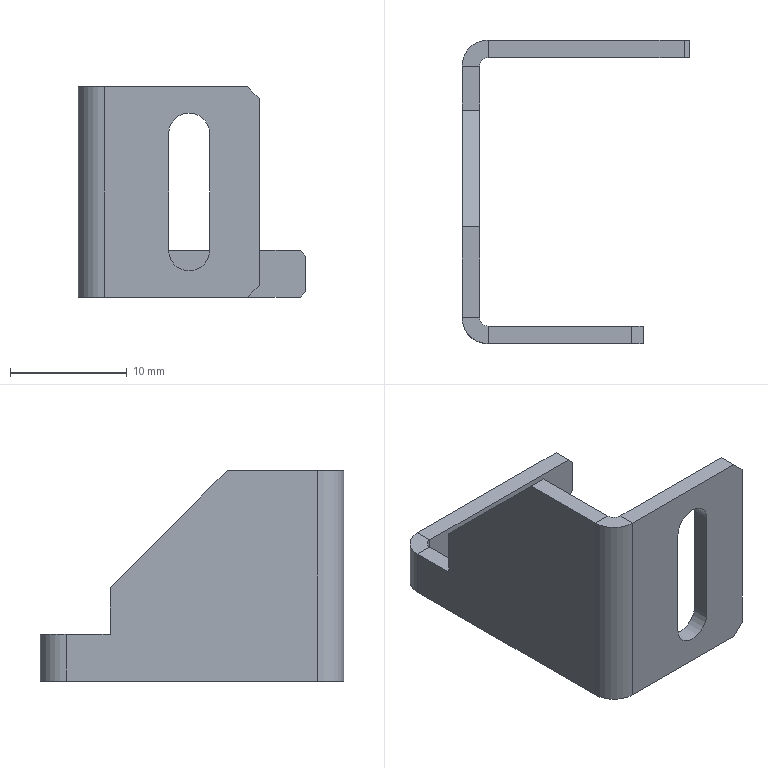Part | SolidWorks | mm | 1 solid | 34 faces | box 19.5 x 26 x 18 mm | volume 897 mm3 | plane 27 | cylinder 7 | commonest cylinder face diameters 3.5 x3 1.473 x2 4.473 x2
Drawing notes:
BOTH 90° BENDS: INSIDE R0.74, OUTSIDE R2.24 (1.5 THK) | from the solid: Z-axis cylinders dia 1.473 and 4.473 at (x2.24,y2.24) L18 and (x2.24,y23.76) L4; wall planes x0/x1.5 give 1.5 thk
2X C1 AT 15.50 FLANGE END, BOTH CORNERS (Z=0 & Z=18) | from the solid: Two inclined planes 45deg, size 1.0x1.5x1.0, at bbox_from [14.5,0,0] and [14.5,0,17] on the x=15.5 flange face (y 0-1.5, z 1-17)
STEP:
#1=CARTESIAN_POINT('',(8.,-1.5,15.75));
#2=VERTEX_POINT('',#1);
#3=CARTESIAN_POINT('',(9.75,-1.5,14.));
#4=VERTEX_POINT('',#3);
#5=CARTESIAN_POINT('',(8.,-1.5,14.));
#6=DIRECTION('',(0.,1.,0.));
#7=DIRECTION('',(0.,0.,1.));
#8=AXIS2_PLACEMENT_3D('',#5,#6,#7);
#9=CIRCLE('',#8,1.75);
#10=EDGE_CURVE('',#2,#4,#9,.T.);
#11=ORIENTED_EDGE('',*,*,#10,.F.);
#12=CARTESIAN_POINT('',(8.,0.,15.75));
#13=VERTEX_POINT('',#12);
#14=CARTESIAN_POINT('',(8.,-26.,15.75));
#15=DIRECTION('',(0.,1.,0.));
#16=VECTOR('',#15,1000.);
#17=LINE('',#14,#16);
#18=EDGE_CURVE('',#2,#13,#17,.T.);
#19=ORIENTED_EDGE('',*,*,#18,.T.);
#20=CARTESIAN_POINT('',(9.75,0.,14.));
#21=VERTEX_POINT('',#20);
#22=CARTESIAN_POINT('',(8.,0.,14.));
#23=DIRECTION('',(0.,1.,0.));
#24=DIRECTION('',(0.,0.,1.));
#25=AXIS2_PLACEMENT_3D('',#22,#23,#24);
#26=CIRCLE('',#25,1.75);
#27=EDGE_CURVE('',#13,#21,#26,.T.);
#28=ORIENTED_EDGE('',*,*,#27,.T.);
#29=CARTESIAN_POINT('',(9.75,-26.,14.));
#30=DIRECTION('',(0.,1.,0.));
#31=VECTOR('',#30,1000.);
#32=LINE('',#29,#31);
#33=EDGE_CURVE('',#4,#21,#32,.T.);
#34=ORIENTED_EDGE('',*,*,#33,.F.);
#35=EDGE_LOOP('',(#11,#19,#28,#34));
#36=FACE_OUTER_BOUND('',#35,.T.);
#37=CARTESIAN_POINT('',(8.,-26.,14.));
#38=DIRECTION('',(0.,1.,0.));
#39=DIRECTION('',(0.,0.,1.));
#40=AXIS2_PLACEMENT_3D('',#37,#38,#39);
#41=CYLINDRICAL_SURFACE('',#40,1.75);
#42=ADVANCED_FACE('',(#36),#41,.F.);
#43=CARTESIAN_POINT('',(0.7366,23.,4.));
#44=VERTEX_POINT('',#43);
#45=CARTESIAN_POINT('',(17.5,23.,4.));
#46=VERTEX_POINT('',#45);
#47=CARTESIAN_POINT('',(18.,23.,4.));
#48=DIRECTION('',(1.,0.,0.));
#49=VECTOR('',#48,1000.);
#50=LINE('',#47,#49);
#51=EDGE_CURVE('',#44,#46,#50,.T.);
#52=ORIENTED_EDGE('',*,*,#51,.T.);
#53=CARTESIAN_POINT('',(17.5,24.5,4.));
#54=VERTEX_POINT('',#53);
#55=CARTESIAN_POINT('',(17.5,24.5,4.));
#56=DIRECTION('',(0.,1.,0.));
#57=VECTOR('',#56,1000.);
#58=LINE('',#55,#57);
#59=EDGE_CURVE('',#46,#54,#58,.T.);
#60=ORIENTED_EDGE('',*,*,#59,.T.);
#61=CARTESIAN_POINT('',(0.7366,24.5,4.));
#62=VERTEX_POINT('',#61);
#63=CARTESIAN_POINT('',(18.,24.5,4.));
#64=DIRECTION('',(1.,0.,0.));
#65=VECTOR('',#64,1000.);
#66=LINE('',#63,#65);
#67=EDGE_CURVE('',#62,#54,#66,.T.);
#68=ORIENTED_EDGE('',*,*,#67,.F.);
#69=CARTESIAN_POINT('',(0.7366,24.5,4.));
#70=DIRECTION('',(-0.,-1.,0.));
#71=VECTOR('',#70,1000.);
#72=LINE('',#69,#71);
#73=EDGE_CURVE('',#62,#44,#72,.T.);
#74=ORIENTED_EDGE('',*,*,#73,.T.);
#75=EDGE_LOOP('',(#52,#60,#68,#74));
#76=FACE_OUTER_BOUND('',#75,.T.);
#77=CARTESIAN_POINT('',(24.5,30.5,4.));
#78=DIRECTION('',(0.,0.,-1.));
#79=DIRECTION('',(-1.,0.,0.));
#80=AXIS2_PLACEMENT_3D('',#77,#78,#79);
#81=PLANE('',#80);
#82=ADVANCED_FACE('',(#76),#81,.F.);
#83=CARTESIAN_POINT('',(0.,18.5,4.));
#84=VERTEX_POINT('',#83);
#85=CARTESIAN_POINT('',(0.,22.263,4.));
#86=VERTEX_POINT('',#85);
#87=CARTESIAN_POINT('',(0.,23.,4.));
#88=DIRECTION('',(0.,1.,0.));
#89=VECTOR('',#88,1000.);
#90=LINE('',#87,#89);
#91=EDGE_CURVE('',#84,#86,#90,.T.);
#92=ORIENTED_EDGE('',*,*,#91,.T.);
#93=CARTESIAN_POINT('',(-1.5,22.263,4.));
#94=VERTEX_POINT('',#93);
#95=CARTESIAN_POINT('',(0.,22.263,4.));
#96=DIRECTION('',(-1.,0.,0.));
#97=VECTOR('',#96,1000.);
#98=LINE('',#95,#97);
#99=EDGE_CURVE('',#86,#94,#98,.T.);
#100=ORIENTED_EDGE('',*,*,#99,.T.);
#101=CARTESIAN_POINT('',(-1.5,18.5,4.));
#102=VERTEX_POINT('',#101);
#103=CARTESIAN_POINT('',(-1.5,23.,4.));
#104=DIRECTION('',(0.,1.,0.));
#105=VECTOR('',#104,1000.);
#106=LINE('',#103,#105);
#107=EDGE_CURVE('',#102,#94,#106,.T.);
#108=ORIENTED_EDGE('',*,*,#107,.F.);
#109=CARTESIAN_POINT('',(24.5,18.5,4.));
#110=DIRECTION('',(-1.,0.,0.));
#111=VECTOR('',#110,1000.);
#112=LINE('',#109,#111);
#113=EDGE_CURVE('',#84,#102,#112,.T.);
#114=ORIENTED_EDGE('',*,*,#113,.F.);
#115=EDGE_LOOP('',(#92,#100,#108,#114));
#116=FACE_OUTER_BOUND('',#115,.T.);
#117=CARTESIAN_POINT('',(24.5,30.5,4.));
#118=DIRECTION('',(0.,0.,-1.));
#119=DIRECTION('',(-1.,0.,0.));
#120=AXIS2_PLACEMENT_3D('',#117,#118,#119);
#121=PLANE('',#120);
#122=ADVANCED_FACE('',(#116),#121,.F.);
#123=CARTESIAN_POINT('',(0.,8.5,18.));
#124=VERTEX_POINT('',#123);
#125=CARTESIAN_POINT('',(0.,0.7366,18.));
#126=VERTEX_POINT('',#125);
#127=CARTESIAN_POINT('',(0.,23.,18.));
#128=DIRECTION('',(-0.,-1.,0.));
#129=VECTOR('',#128,1000.);
#130=LINE('',#127,#129);
#131=EDGE_CURVE('',#124,#126,#130,.T.);
#132=ORIENTED_EDGE('',*,*,#131,.F.);
#133=CARTESIAN_POINT('',(-1.5,8.5,18.));
#134=VERTEX_POINT('',#133);
#135=CARTESIAN_POINT('',(-1.5,8.5,18.));
#136=DIRECTION('',(-1.,0.,0.));
#137=VECTOR('',#136,1000.);
#138=LINE('',#135,#137);
#139=EDGE_CURVE('',#124,#134,#138,.T.);
#140=ORIENTED_EDGE('',*,*,#139,.T.);
#141=CARTESIAN_POINT('',(-1.5,0.7366,18.));
#142=VERTEX_POINT('',#141);
#143=CARTESIAN_POINT('',(-1.5,23.,18.));
#144=DIRECTION('',(-0.,-1.,0.));
#145=VECTOR('',#144,1000.);
#146=LINE('',#143,#145);
#147=EDGE_CURVE('',#134,#142,#146,.T.);
#148=ORIENTED_EDGE('',*,*,#147,.T.);
#149=CARTESIAN_POINT('',(-1.5,0.7366,18.));
#150=DIRECTION('',(1.,-0.,0.));
#151=VECTOR('',#150,1000.);
#152=LINE('',#149,#151);
#153=EDGE_CURVE('',#142,#126,#152,.T.);
#154=ORIENTED_EDGE('',*,*,#153,.T.);
#155=EDGE_LOOP('',(#132,#140,#148,#154));
#156=FACE_OUTER_BOUND('',#155,.T.);
#157=CARTESIAN_POINT('',(0.7366,24.5,18.));
#158=DIRECTION('',(0.,0.,1.));
#159=DIRECTION('',(1.,0.,0.));
#160=AXIS2_PLACEMENT_3D('',#157,#158,#159);
#161=PLANE('',#160);
#162=ADVANCED_FACE('',(#156),#161,.T.);
#163=CARTESIAN_POINT('',(0.7366,23.,0.));
#164=VERTEX_POINT('',#163);
#165=CARTESIAN_POINT('',(0.7366,24.5,0.));
#166=VERTEX_POINT('',#165);
#167=CARTESIAN_POINT('',(0.7366,23.,0.));
#168=DIRECTION('',(0.,1.,0.));
#169=VECTOR('',#168,1000.);
#170=LINE('',#167,#169);
#171=EDGE_CURVE('',#164,#166,#170,.T.);
#172=ORIENTED_EDGE('',*,*,#171,.F.);
#173=CARTESIAN_POINT('',(0.,22.263,0.));
#174=VERTEX_POINT('',#173);
#175=CARTESIAN_POINT('',(0.7366,22.263,0.));
#176=DIRECTION('',(0.,0.,1.));
#177=DIRECTION('',(-1.,0.,0.));
#178=AXIS2_PLACEMENT_3D('',#175,#176,#177);
#179=CIRCLE('',#178,0.7366);
#180=EDGE_CURVE('',#164,#174,#179,.T.);
#181=ORIENTED_EDGE('',*,*,#180,.T.);
#182=CARTESIAN_POINT('',(-1.5,22.263,0.));
#183=VERTEX_POINT('',#182);
#184=CARTESIAN_POINT('',(-1.5,22.263,0.));
#185=DIRECTION('',(1.,0.,0.));
#186=VECTOR('',#185,1000.);
#187=LINE('',#184,#186);
#188=EDGE_CURVE('',#183,#174,#187,.T.);
#189=ORIENTED_EDGE('',*,*,#188,.F.);
#190=CARTESIAN_POINT('',(0.7366,22.263,0.));
#191=DIRECTION('',(0.,0.,1.));
#192=DIRECTION('',(1.,0.,0.));
#193=AXIS2_PLACEMENT_3D('',#190,#191,#192);
#194=CIRCLE('',#193,2.237);
#195=EDGE_CURVE('',#166,#183,#194,.T.);
#196=ORIENTED_EDGE('',*,*,#195,.F.);
#197=EDGE_LOOP('',(#172,#181,#189,#196));
#198=FACE_OUTER_BOUND('',#197,.T.);
#199=CARTESIAN_POINT('',(0.7366,23.,0.));
#200=DIRECTION('',(0.,0.,-1.));
#201=DIRECTION('',(-1.,0.,0.));
#202=AXIS2_PLACEMENT_3D('',#199,#200,#201);
#203=PLANE('',#202);
#204=ADVANCED_FACE('',(#198),#203,.T.);
#205=CARTESIAN_POINT('',(17.5,24.5,0.));
#206=VERTEX_POINT('',#205);
#207=CARTESIAN_POINT('',(18.,24.5,0.));
#208=DIRECTION('',(-1.,0.,0.));
#209=VECTOR('',#208,1000.);
#210=LINE('',#207,#209);
#211=EDGE_CURVE('',#206,#166,#210,.T.);
#212=ORIENTED_EDGE('',*,*,#211,.F.);
#213=CARTESIAN_POINT('',(17.5,23.,0.));
#214=VERTEX_POINT('',#213);
#215=CARTESIAN_POINT('',(17.5,22.263,0.));
#216=DIRECTION('',(0.,-1.,0.));
#217=VECTOR('',#216,1000.);
#218=LINE('',#215,#217);
#219=EDGE_CURVE('',#206,#214,#218,.T.);
#220=ORIENTED_EDGE('',*,*,#219,.T.);
#221=CARTESIAN_POINT('',(18.,23.,0.));
#222=DIRECTION('',(-1.,0.,0.));
#223=VECTOR('',#222,1000.);
#224=LINE('',#221,#223);
#225=EDGE_CURVE('',#214,#164,#224,.T.);
#226=ORIENTED_EDGE('',*,*,#225,.T.);
#227=ORIENTED_EDGE('',*,*,#171,.T.);
#228=EDGE_LOOP('',(#212,#220,#226,#227));
#229=FACE_OUTER_BOUND('',#228,.T.);
#230=CARTESIAN_POINT('',(-1.5,22.263,0.));
#231=DIRECTION('',(0.,0.,-1.));
#232=DIRECTION('',(-1.,0.,0.));
#233=AXIS2_PLACEMENT_3D('',#230,#231,#232);
#234=PLANE('',#233);
#235=ADVANCED_FACE('',(#229),#234,.T.);
#236=CARTESIAN_POINT('',(0.7366,0.,18.));
#237=VERTEX_POINT('',#236);
#238=CARTESIAN_POINT('',(0.7366,-1.5,18.));
#239=VERTEX_POINT('',#238);
#240=CARTESIAN_POINT('',(0.7366,0.,18.));
#241=DIRECTION('',(0.,-1.,0.));
#242=VECTOR('',#241,1000.);
#243=LINE('',#240,#242);
#244=EDGE_CURVE('',#237,#239,#243,.T.);
#245=ORIENTED_EDGE('',*,*,#244,.F.);
#246=CARTESIAN_POINT('',(0.7366,0.7366,18.));
#247=DIRECTION('',(0.,0.,1.));
#248=DIRECTION('',(-1.,0.,0.));
#249=AXIS2_PLACEMENT_3D('',#246,#247,#248);
#250=CIRCLE('',#249,0.7366);
#251=EDGE_CURVE('',#126,#237,#250,.T.);
#252=ORIENTED_EDGE('',*,*,#251,.F.);
#253=ORIENTED_EDGE('',*,*,#153,.F.);
#254=CARTESIAN_POINT('',(0.7366,0.7366,18.));
#255=DIRECTION('',(0.,0.,1.));
#256=DIRECTION('',(1.,0.,0.));
#257=AXIS2_PLACEMENT_3D('',#254,#255,#256);
#258=CIRCLE('',#257,2.237);
#259=EDGE_CURVE('',#142,#239,#258,.T.);
#260=ORIENTED_EDGE('',*,*,#259,.T.);
#261=EDGE_LOOP('',(#245,#252,#253,#260));
#262=FACE_OUTER_BOUND('',#261,.T.);
#263=CARTESIAN_POINT('',(0.7366,0.,18.));
#264=DIRECTION('',(0.,0.,1.));
#265=DIRECTION('',(1.,0.,0.));
#266=AXIS2_PLACEMENT_3D('',#263,#264,#265);
#267=PLANE('',#266);
#268=ADVANCED_FACE('',(#262),#267,.T.);
#269=CARTESIAN_POINT('',(13.,-1.5,18.));
#270=VERTEX_POINT('',#269);
#271=CARTESIAN_POINT('',(0.,-1.5,18.));
#272=DIRECTION('',(1.,0.,0.));
#273=VECTOR('',#272,1000.);
#274=LINE('',#271,#273);
#275=EDGE_CURVE('',#239,#270,#274,.T.);
#276=ORIENTED_EDGE('',*,*,#275,.T.);
#277=CARTESIAN_POINT('',(13.,0.,18.));
#278=VERTEX_POINT('',#277);
#279=CARTESIAN_POINT('',(13.,0.7366,18.));
#280=DIRECTION('',(0.,1.,0.));
#281=VECTOR('',#280,1000.);
#282=LINE('',#279,#281);
#283=EDGE_CURVE('',#270,#278,#282,.T.);
#284=ORIENTED_EDGE('',*,*,#283,.T.);
#285=CARTESIAN_POINT('',(0.,0.,18.));
#286=DIRECTION('',(1.,0.,0.));
#287=VECTOR('',#286,1000.);
#288=LINE('',#285,#287);
#289=EDGE_CURVE('',#237,#278,#288,.T.);
#290=ORIENTED_EDGE('',*,*,#289,.F.);
#291=ORIENTED_EDGE('',*,*,#244,.T.);
#292=EDGE_LOOP('',(#276,#284,#290,#291));
#293=FACE_OUTER_BOUND('',#292,.T.);
#294=CARTESIAN_POINT('',(-1.5,0.7366,18.));
#295=DIRECTION('',(0.,0.,1.));
#296=DIRECTION('',(1.,0.,0.));
#297=AXIS2_PLACEMENT_3D('',#294,#295,#296);
#298=PLANE('',#297);
#299=ADVANCED_FACE('',(#293),#298,.T.);
#300=CARTESIAN_POINT('',(0.,0.7366,0.));
#301=VERTEX_POINT('',#300);
#302=CARTESIAN_POINT('',(-1.5,0.7366,0.));
#303=VERTEX_POINT('',#302);
#304=CARTESIAN_POINT('',(0.,0.7366,0.));
#305=DIRECTION('',(-1.,0.,0.));
#306=VECTOR('',#305,1000.);
#307=LINE('',#304,#306);
#308=EDGE_CURVE('',#301,#303,#307,.T.);
#309=ORIENTED_EDGE('',*,*,#308,.F.);
#310=CARTESIAN_POINT('',(0.7366,0.,0.));
#311=VERTEX_POINT('',#310);
#312=CARTESIAN_POINT('',(0.7366,0.7366,0.));
#313=DIRECTION('',(0.,0.,1.));
#314=DIRECTION('',(-1.,0.,0.));
#315=AXIS2_PLACEMENT_3D('',#312,#313,#314);
#316=CIRCLE('',#315,0.7366);
#317=EDGE_CURVE('',#301,#311,#316,.T.);
#318=ORIENTED_EDGE('',*,*,#317,.T.);
#319=CARTESIAN_POINT('',(0.7366,-1.5,0.));
#320=VERTEX_POINT('',#319);
#321=CARTESIAN_POINT('',(0.7366,-1.5,0.));
#322=DIRECTION('',(0.,1.,0.));
#323=VECTOR('',#322,1000.);
#324=LINE('',#321,#323);
#325=EDGE_CURVE('',#320,#311,#324,.T.);
#326=ORIENTED_EDGE('',*,*,#325,.F.);
#327=CARTESIAN_POINT('',(0.7366,0.7366,0.));
#328=DIRECTION('',(0.,0.,1.));
#329=DIRECTION('',(1.,0.,0.));
#330=AXIS2_PLACEMENT_3D('',#327,#328,#329);
#331=CIRCLE('',#330,2.237);
#332=EDGE_CURVE('',#303,#320,#331,.T.);
#333=ORIENTED_EDGE('',*,*,#332,.F.);
#334=EDGE_LOOP('',(#309,#318,#326,#333));
#335=FACE_OUTER_BOUND('',#334,.T.);
#336=CARTESIAN_POINT('',(0.,0.7366,0.));
#337=DIRECTION('',(0.,0.,-1.));
#338=DIRECTION('',(-1.,0.,0.));
#339=AXIS2_PLACEMENT_3D('',#336,#337,#338);
#340=PLANE('',#339);
#341=ADVANCED_FACE('',(#335),#340,.T.);
#342=CARTESIAN_POINT('',(0.,23.,0.));
#343=DIRECTION('',(-0.,-1.,0.));
#344=VECTOR('',#343,1000.);
#345=LINE('',#342,#344);
#346=EDGE_CURVE('',#174,#301,#345,.T.);
#347=ORIENTED_EDGE('',*,*,#346,.T.);
#348=ORIENTED_EDGE('',*,*,#308,.T.);
#349=CARTESIAN_POINT('',(-1.5,23.,0.));
#350=DIRECTION('',(-0.,-1.,0.));
#351=VECTOR('',#350,1000.);
#352=LINE('',#349,#351);
#353=EDGE_CURVE('',#183,#303,#352,.T.);
#354=ORIENTED_EDGE('',*,*,#353,.F.);
#355=ORIENTED_EDGE('',*,*,#188,.T.);
#356=EDGE_LOOP('',(#347,#348,#354,#355));
#357=FACE_OUTER_BOUND('',#356,.T.);
#358=CARTESIAN_POINT('',(0.7366,-1.5,0.));
#359=DIRECTION('',(0.,0.,-1.));
#360=DIRECTION('',(-1.,0.,0.));
#361=AXIS2_PLACEMENT_3D('',#358,#359,#360);
#362=PLANE('',#361);
#363=ADVANCED_FACE('',(#357),#362,.T.);
#364=CARTESIAN_POINT('',(6.25,-1.5,4.));
#365=VERTEX_POINT('',#364);
#366=CARTESIAN_POINT('',(6.25,-1.5,14.));
#367=VERTEX_POINT('',#366);
#368=CARTESIAN_POINT('',(6.25,-1.5,18.));
#369=DIRECTION('',(0.,0.,1.));
#370=VECTOR('',#369,1000.);
#371=LINE('',#368,#370);
#372=EDGE_CURVE('',#365,#367,#371,.T.);
#373=ORIENTED_EDGE('',*,*,#372,.T.);
#374=CARTESIAN_POINT('',(8.,-1.5,14.));
#375=DIRECTION('',(0.,1.,0.));
#376=DIRECTION('',(0.,0.,1.));
#377=AXIS2_PLACEMENT_3D('',#374,#375,#376);
#378=CIRCLE('',#377,1.75);
#379=EDGE_CURVE('',#367,#2,#378,.T.);
#380=ORIENTED_EDGE('',*,*,#379,.T.);
#381=ORIENTED_EDGE('',*,*,#10,.T.);
#382=CARTESIAN_POINT('',(9.75,-1.5,4.));
#383=VERTEX_POINT('',#382);
#384=CARTESIAN_POINT('',(9.75,-1.5,18.));
#385=DIRECTION('',(0.,0.,-1.));
#386=VECTOR('',#385,1000.);
#387=LINE('',#384,#386);
#388=EDGE_CURVE('',#4,#383,#387,.T.);
#389=ORIENTED_EDGE('',*,*,#388,.T.);
#390=CARTESIAN_POINT('',(8.,-1.5,4.));
#391=DIRECTION('',(0.,1.,0.));
#392=DIRECTION('',(0.,0.,1.));
#393=AXIS2_PLACEMENT_3D('',#390,#391,#392);
#394=CIRCLE('',#393,1.75);
#395=EDGE_CURVE('',#383,#365,#394,.T.);
#396=ORIENTED_EDGE('',*,*,#395,.T.);
#397=EDGE_LOOP('',(#373,#380,#381,#389,#396));
#398=FACE_BOUND('',#397,.T.);
#399=CARTESIAN_POINT('',(13.,-1.5,0.));
#400=VERTEX_POINT('',#399);
#401=CARTESIAN_POINT('',(0.,-1.5,0.));
#402=DIRECTION('',(1.,0.,0.));
#403=VECTOR('',#402,1000.);
#404=LINE('',#401,#403);
#405=EDGE_CURVE('',#320,#400,#404,.T.);
#406=ORIENTED_EDGE('',*,*,#405,.T.);
#407=CARTESIAN_POINT('',(14.,-1.5,1.));
#408=VERTEX_POINT('',#407);
#409=CARTESIAN_POINT('',(13.,-1.5,0.));
#410=DIRECTION('',(0.7071,0.,0.7071));
#411=VECTOR('',#410,1000.);
#412=LINE('',#409,#411);
#413=EDGE_CURVE('',#400,#408,#412,.T.);
#414=ORIENTED_EDGE('',*,*,#413,.T.);
#415=CARTESIAN_POINT('',(14.,-1.5,17.));
#416=VERTEX_POINT('',#415);
#417=CARTESIAN_POINT('',(14.,-1.5,18.));
#418=DIRECTION('',(0.,0.,-1.));
#419=VECTOR('',#418,1000.);
#420=LINE('',#417,#419);
#421=EDGE_CURVE('',#416,#408,#420,.T.);
#422=ORIENTED_EDGE('',*,*,#421,.F.);
#423=CARTESIAN_POINT('',(14.,-1.5,17.));
#424=DIRECTION('',(-0.7071,0.,0.7071));
#425=VECTOR('',#424,1000.);
#426=LINE('',#423,#425);
#427=EDGE_CURVE('',#416,#270,#426,.T.);
#428=ORIENTED_EDGE('',*,*,#427,.T.);
#429=ORIENTED_EDGE('',*,*,#275,.F.);
#430=CARTESIAN_POINT('',(0.7366,-1.5,18.));
#431=DIRECTION('',(0.,0.,-1.));
#432=VECTOR('',#431,1000.);
#433=LINE('',#430,#432);
#434=EDGE_CURVE('',#239,#320,#433,.T.);
#435=ORIENTED_EDGE('',*,*,#434,.T.);
#436=EDGE_LOOP('',(#406,#414,#422,#428,#429,#435));
#437=FACE_OUTER_BOUND('',#436,.T.);
#438=CARTESIAN_POINT('',(0.,-1.5,18.));
#439=DIRECTION('',(0.,1.,0.));
#440=DIRECTION('',(0.,0.,1.));
#441=AXIS2_PLACEMENT_3D('',#438,#439,#440);
#442=PLANE('',#441);
#443=ADVANCED_FACE('',(#398,#437),#442,.F.);
#444=ORIENTED_EDGE('',*,*,#421,.T.);
#445=CARTESIAN_POINT('',(14.,0.,1.));
#446=VERTEX_POINT('',#445);
#447=CARTESIAN_POINT('',(14.,0.,1.));
#448=DIRECTION('',(0.,1.,0.));
#449=VECTOR('',#448,1000.);
#450=LINE('',#447,#449);
#451=EDGE_CURVE('',#408,#446,#450,.T.);
#452=ORIENTED_EDGE('',*,*,#451,.T.);
#453=CARTESIAN_POINT('',(14.,0.,17.));
#454=VERTEX_POINT('',#453);
#455=CARTESIAN_POINT('',(14.,0.,18.));
#456=DIRECTION('',(0.,0.,-1.));
#457=VECTOR('',#456,1000.);
#458=LINE('',#455,#457);
#459=EDGE_CURVE('',#454,#446,#458,.T.);
#460=ORIENTED_EDGE('',*,*,#459,.F.);
#461=CARTESIAN_POINT('',(14.,0.,17.));
#462=DIRECTION('',(0.,-1.,0.));
#463=VECTOR('',#462,1000.);
#464=LINE('',#461,#463);
#465=EDGE_CURVE('',#454,#416,#464,.T.);
#466=ORIENTED_EDGE('',*,*,#465,.T.);
#467=EDGE_LOOP('',(#444,#452,#460,#466));
#468=FACE_OUTER_BOUND('',#467,.T.);
#469=CARTESIAN_POINT('',(14.,0.,18.));
#470=DIRECTION('',(1.,0.,0.));
#471=DIRECTION('',(0.,0.,-1.));
#472=AXIS2_PLACEMENT_3D('',#469,#470,#471);
#473=PLANE('',#472);
#474=ADVANCED_FACE('',(#468),#473,.T.);
#475=CARTESIAN_POINT('',(6.25,0.,14.));
#476=VERTEX_POINT('',#475);
#477=CARTESIAN_POINT('',(8.,0.,14.));
#478=DIRECTION('',(0.,1.,0.));
#479=DIRECTION('',(0.,0.,1.));
#480=AXIS2_PLACEMENT_3D('',#477,#478,#479);
#481=CIRCLE('',#480,1.75);
#482=EDGE_CURVE('',#476,#13,#481,.T.);
#483=ORIENTED_EDGE('',*,*,#482,.F.);
#484=CARTESIAN_POINT('',(6.25,0.,4.));
#485=VERTEX_POINT('',#484);
#486=CARTESIAN_POINT('',(6.25,0.,14.));
#487=DIRECTION('',(0.,0.,1.));
#488=VECTOR('',#487,1000.);
#489=LINE('',#486,#488);
#490=EDGE_CURVE('',#485,#476,#489,.T.);
#491=ORIENTED_EDGE('',*,*,#490,.F.);
#492=CARTESIAN_POINT('',(9.75,0.,4.));
#493=VERTEX_POINT('',#492);
#494=CARTESIAN_POINT('',(8.,0.,4.));
#495=DIRECTION('',(0.,1.,0.));
#496=DIRECTION('',(0.,0.,1.));
#497=AXIS2_PLACEMENT_3D('',#494,#495,#496);
#498=CIRCLE('',#497,1.75);
#499=EDGE_CURVE('',#493,#485,#498,.T.);
#500=ORIENTED_EDGE('',*,*,#499,.F.);
#501=CARTESIAN_POINT('',(9.75,0.,14.));
#502=DIRECTION('',(0.,0.,-1.));
#503=VECTOR('',#502,1000.);
#504=LINE('',#501,#503);
#505=EDGE_CURVE('',#21,#493,#504,.T.);
#506=ORIENTED_EDGE('',*,*,#505,.F.);
#507=ORIENTED_EDGE('',*,*,#27,.F.);
#508=EDGE_LOOP('',(#483,#491,#500,#506,#507));
#509=FACE_BOUND('',#508,.T.);
#510=ORIENTED_EDGE('',*,*,#459,.T.);
#511=CARTESIAN_POINT('',(13.,0.,0.));
#512=VERTEX_POINT('',#511);
#513=CARTESIAN_POINT('',(15.5,0.,2.5));
#514=DIRECTION('',(-0.7071,0.,-0.7071));
#515=VECTOR('',#514,1000.);
#516=LINE('',#513,#515);
#517=EDGE_CURVE('',#446,#512,#516,.T.);
#518=ORIENTED_EDGE('',*,*,#517,.T.);
#519=CARTESIAN_POINT('',(0.,0.,0.));
#520=DIRECTION('',(1.,0.,0.));
#521=VECTOR('',#520,1000.);
#522=LINE('',#519,#521);
#523=EDGE_CURVE('',#311,#512,#522,.T.);
#524=ORIENTED_EDGE('',*,*,#523,.F.);
#525=CARTESIAN_POINT('',(0.7366,0.,18.));
#526=DIRECTION('',(0.,0.,-1.));
#527=VECTOR('',#526,1000.);
#528=LINE('',#525,#527);
#529=EDGE_CURVE('',#237,#311,#528,.T.);
#530=ORIENTED_EDGE('',*,*,#529,.F.);
#531=ORIENTED_EDGE('',*,*,#289,.T.);
#532=CARTESIAN_POINT('',(6.5,0.,24.5));
#533=DIRECTION('',(0.7071,0.,-0.7071));
#534=VECTOR('',#533,1000.);
#535=LINE('',#532,#534);
#536=EDGE_CURVE('',#278,#454,#535,.T.);
#537=ORIENTED_EDGE('',*,*,#536,.T.);
#538=EDGE_LOOP('',(#510,#518,#524,#530,#531,#537));
#539=FACE_OUTER_BOUND('',#538,.T.);
#540=CARTESIAN_POINT('',(0.,0.,18.));
#541=DIRECTION('',(0.,1.,0.));
#542=DIRECTION('',(0.,0.,1.));
#543=AXIS2_PLACEMENT_3D('',#540,#541,#542);
#544=PLANE('',#543);
#545=ADVANCED_FACE('',(#509,#539),#544,.T.);
#546=ORIENTED_EDGE('',*,*,#317,.F.);
#547=CARTESIAN_POINT('',(0.,0.7366,18.));
#548=DIRECTION('',(0.,0.,-1.));
#549=VECTOR('',#548,1000.);
#550=LINE('',#547,#549);
#551=EDGE_CURVE('',#126,#301,#550,.T.);
#552=ORIENTED_EDGE('',*,*,#551,.F.);
#553=ORIENTED_EDGE('',*,*,#251,.T.);
#554=ORIENTED_EDGE('',*,*,#529,.T.);
#555=EDGE_LOOP('',(#546,#552,#553,#554));
#556=FACE_OUTER_BOUND('',#555,.T.);
#557=CARTESIAN_POINT('',(0.7366,0.7366,18.));
#558=DIRECTION('',(0.,0.,-1.));
#559=DIRECTION('',(-1.,0.,0.));
#560=AXIS2_PLACEMENT_3D('',#557,#558,#559);
#561=CYLINDRICAL_SURFACE('',#560,0.7366);
#562=ADVANCED_FACE('',(#556),#561,.F.);
#563=CARTESIAN_POINT('',(0.,18.5,8.));
#564=VERTEX_POINT('',#563);
#565=CARTESIAN_POINT('',(0.,18.5,18.));
#566=DIRECTION('',(0.,0.,-1.));
#567=VECTOR('',#566,1000.);
#568=LINE('',#565,#567);
#569=EDGE_CURVE('',#564,#84,#568,.T.);
#570=ORIENTED_EDGE('',*,*,#569,.F.);
#571=CARTESIAN_POINT('',(0.,15.75,10.75));
#572=DIRECTION('',(-0.,-0.7071,0.7071));
#573=VECTOR('',#572,1000.);
#574=LINE('',#571,#573);
#575=EDGE_CURVE('',#564,#124,#574,.T.);
#576=ORIENTED_EDGE('',*,*,#575,.T.);
#577=ORIENTED_EDGE('',*,*,#131,.T.);
#578=ORIENTED_EDGE('',*,*,#551,.T.);
#579=ORIENTED_EDGE('',*,*,#346,.F.);
#580=CARTESIAN_POINT('',(0.,22.263,18.));
#581=DIRECTION('',(0.,0.,-1.));
#582=VECTOR('',#581,1000.);
#583=LINE('',#580,#582);
#584=EDGE_CURVE('',#86,#174,#583,.T.);
#585=ORIENTED_EDGE('',*,*,#584,.F.);
#586=ORIENTED_EDGE('',*,*,#91,.F.);
#587=EDGE_LOOP('',(#570,#576,#577,#578,#579,#585,#586));
#588=FACE_OUTER_BOUND('',#587,.T.);
#589=CARTESIAN_POINT('',(0.,23.,18.));
#590=DIRECTION('',(1.,-0.,0.));
#591=DIRECTION('',(0.,1.,0.));
#592=AXIS2_PLACEMENT_3D('',#589,#590,#591);
#593=PLANE('',#592);
#594=ADVANCED_FACE('',(#588),#593,.T.);
#595=CARTESIAN_POINT('',(0.7366,22.263,4.));
#596=DIRECTION('',(0.,0.,-1.));
#597=DIRECTION('',(-1.,0.,0.));
#598=AXIS2_PLACEMENT_3D('',#595,#596,#597);
#599=CIRCLE('',#598,0.7366);
#600=EDGE_CURVE('',#86,#44,#599,.T.);
#601=ORIENTED_EDGE('',*,*,#600,.F.);
#602=ORIENTED_EDGE('',*,*,#584,.T.);
#603=ORIENTED_EDGE('',*,*,#180,.F.);
#604=CARTESIAN_POINT('',(0.7366,23.,18.));
#605=DIRECTION('',(0.,0.,-1.));
#606=VECTOR('',#605,1000.);
#607=LINE('',#604,#606);
#608=EDGE_CURVE('',#44,#164,#607,.T.);
#609=ORIENTED_EDGE('',*,*,#608,.F.);
#610=EDGE_LOOP('',(#601,#602,#603,#609));
#611=FACE_OUTER_BOUND('',#610,.T.);
#612=CARTESIAN_POINT('',(0.7366,22.263,18.));
#613=DIRECTION('',(0.,0.,-1.));
#614=DIRECTION('',(-1.,0.,0.));
#615=AXIS2_PLACEMENT_3D('',#612,#613,#614);
#616=CYLINDRICAL_SURFACE('',#615,0.7366);
#617=ADVANCED_FACE('',(#611),#616,.F.);
#618=CARTESIAN_POINT('',(18.,23.,3.5));
#619=VERTEX_POINT('',#618);
#620=CARTESIAN_POINT('',(18.,23.,0.5));
#621=VERTEX_POINT('',#620);
#622=CARTESIAN_POINT('',(18.,23.,18.));
#623=DIRECTION('',(0.,0.,-1.));
#624=VECTOR('',#623,1000.);
#625=LINE('',#622,#624);
#626=EDGE_CURVE('',#619,#621,#625,.T.);
#627=ORIENTED_EDGE('',*,*,#626,.F.);
#628=CARTESIAN_POINT('',(10.75,23.,10.75));
#629=DIRECTION('',(-0.7071,0.,0.7071));
#630=VECTOR('',#629,1000.);
#631=LINE('',#628,#630);
#632=EDGE_CURVE('',#619,#46,#631,.T.);
#633=ORIENTED_EDGE('',*,*,#632,.T.);
#634=ORIENTED_EDGE('',*,*,#51,.F.);
#635=ORIENTED_EDGE('',*,*,#608,.T.);
#636=ORIENTED_EDGE('',*,*,#225,.F.);
#637=CARTESIAN_POINT('',(26.75,23.,9.25));
#638=DIRECTION('',(0.7071,0.,0.7071));
#639=VECTOR('',#638,1000.);
#640=LINE('',#637,#639);
#641=EDGE_CURVE('',#214,#621,#640,.T.);
#642=ORIENTED_EDGE('',*,*,#641,.T.);
#643=EDGE_LOOP('',(#627,#633,#634,#635,#636,#642));
#644=FACE_OUTER_BOUND('',#643,.T.);
#645=CARTESIAN_POINT('',(18.,23.,18.));
#646=DIRECTION('',(0.,-1.,0.));
#647=DIRECTION('',(0.,0.,-1.));
#648=AXIS2_PLACEMENT_3D('',#645,#646,#647);
#649=PLANE('',#648);
#650=ADVANCED_FACE('',(#644),#649,.T.);
#651=CARTESIAN_POINT('',(18.,24.5,3.5));
#652=VERTEX_POINT('',#651);
#653=CARTESIAN_POINT('',(18.,24.5,0.5));
#654=VERTEX_POINT('',#653);
#655=CARTESIAN_POINT('',(18.,24.5,18.));
#656=DIRECTION('',(0.,0.,-1.));
#657=VECTOR('',#656,1000.);
#658=LINE('',#655,#657);
#659=EDGE_CURVE('',#652,#654,#658,.T.);
#660=ORIENTED_EDGE('',*,*,#659,.F.);
#661=CARTESIAN_POINT('',(18.,23.,3.5));
#662=DIRECTION('',(0.,-1.,0.));
#663=VECTOR('',#662,1000.);
#664=LINE('',#661,#663);
#665=EDGE_CURVE('',#652,#619,#664,.T.);
#666=ORIENTED_EDGE('',*,*,#665,.T.);
#667=ORIENTED_EDGE('',*,*,#626,.T.);
#668=CARTESIAN_POINT('',(18.,24.5,0.5));
#669=DIRECTION('',(0.,1.,0.));
#670=VECTOR('',#669,1000.);
#671=LINE('',#668,#670);
#672=EDGE_CURVE('',#621,#654,#671,.T.);
#673=ORIENTED_EDGE('',*,*,#672,.T.);
#674=EDGE_LOOP('',(#660,#666,#667,#673));
#675=FACE_OUTER_BOUND('',#674,.T.);
#676=CARTESIAN_POINT('',(18.,24.5,18.));
#677=DIRECTION('',(1.,0.,0.));
#678=DIRECTION('',(0.,0.,-1.));
#679=AXIS2_PLACEMENT_3D('',#676,#677,#678);
#680=PLANE('',#679);
#681=ADVANCED_FACE('',(#675),#680,.T.);
#682=ORIENTED_EDGE('',*,*,#67,.T.);
#683=CARTESIAN_POINT('',(17.5,24.5,4.));
#684=DIRECTION('',(0.7071,0.,-0.7071));
#685=VECTOR('',#684,1000.);
#686=LINE('',#683,#685);
#687=EDGE_CURVE('',#54,#652,#686,.T.);
#688=ORIENTED_EDGE('',*,*,#687,.T.);
#689=ORIENTED_EDGE('',*,*,#659,.T.);
#690=CARTESIAN_POINT('',(17.5,24.5,0.));
#691=DIRECTION('',(-0.7071,0.,-0.7071));
#692=VECTOR('',#691,1000.);
#693=LINE('',#690,#692);
#694=EDGE_CURVE('',#654,#206,#693,.T.);
#695=ORIENTED_EDGE('',*,*,#694,.T.);
#696=ORIENTED_EDGE('',*,*,#211,.T.);
#697=CARTESIAN_POINT('',(0.7366,24.5,18.));
#698=DIRECTION('',(0.,0.,-1.));
#699=VECTOR('',#698,1000.);
#700=LINE('',#697,#699);
#701=EDGE_CURVE('',#62,#166,#700,.T.);
#702=ORIENTED_EDGE('',*,*,#701,.F.);
#703=EDGE_LOOP('',(#682,#688,#689,#695,#696,#702));
#704=FACE_OUTER_BOUND('',#703,.T.);
#705=CARTESIAN_POINT('',(18.,24.5,18.));
#706=DIRECTION('',(0.,-1.,0.));
#707=DIRECTION('',(0.,0.,-1.));
#708=AXIS2_PLACEMENT_3D('',#705,#706,#707);
#709=PLANE('',#708);
#710=ADVANCED_FACE('',(#704),#709,.F.);
#711=CARTESIAN_POINT('',(-1.5,22.263,18.));
#712=DIRECTION('',(0.,0.,-1.));
#713=VECTOR('',#712,1000.);
#714=LINE('',#711,#713);
#715=EDGE_CURVE('',#94,#183,#714,.T.);
#716=ORIENTED_EDGE('',*,*,#715,.F.);
#717=CARTESIAN_POINT('',(0.7366,22.263,4.));
#718=DIRECTION('',(0.,0.,-1.));
#719=DIRECTION('',(-1.,0.,0.));
#720=AXIS2_PLACEMENT_3D('',#717,#718,#719);
#721=CIRCLE('',#720,2.237);
#722=EDGE_CURVE('',#94,#62,#721,.T.);
#723=ORIENTED_EDGE('',*,*,#722,.T.);
#724=ORIENTED_EDGE('',*,*,#701,.T.);
#725=ORIENTED_EDGE('',*,*,#195,.T.);
#726=EDGE_LOOP('',(#716,#723,#724,#725));
#727=FACE_OUTER_BOUND('',#726,.T.);
#728=CARTESIAN_POINT('',(0.7366,22.263,18.));
#729=DIRECTION('',(0.,0.,-1.));
#730=DIRECTION('',(-1.,0.,0.));
#731=AXIS2_PLACEMENT_3D('',#728,#729,#730);
#732=CYLINDRICAL_SURFACE('',#731,2.237);
#733=ADVANCED_FACE('',(#727),#732,.T.);
#734=ORIENTED_EDGE('',*,*,#147,.F.);
#735=CARTESIAN_POINT('',(-1.5,18.5,8.));
#736=VERTEX_POINT('',#735);
#737=CARTESIAN_POINT('',(-1.5,18.5,8.));
#738=DIRECTION('',(0.,0.7071,-0.7071));
#739=VECTOR('',#738,1000.);
#740=LINE('',#737,#739);
#741=EDGE_CURVE('',#134,#736,#740,.T.);
#742=ORIENTED_EDGE('',*,*,#741,.T.);
#743=CARTESIAN_POINT('',(-1.5,18.5,32.));
#744=DIRECTION('',(0.,0.,1.));
#745=VECTOR('',#744,1000.);
#746=LINE('',#743,#745);
#747=EDGE_CURVE('',#102,#736,#746,.T.);
#748=ORIENTED_EDGE('',*,*,#747,.F.);
#749=ORIENTED_EDGE('',*,*,#107,.T.);
#750=ORIENTED_EDGE('',*,*,#715,.T.);
#751=ORIENTED_EDGE('',*,*,#353,.T.);
#752=CARTESIAN_POINT('',(-1.5,0.7366,18.));
#753=DIRECTION('',(0.,0.,-1.));
#754=VECTOR('',#753,1000.);
#755=LINE('',#752,#754);
#756=EDGE_CURVE('',#142,#303,#755,.T.);
#757=ORIENTED_EDGE('',*,*,#756,.F.);
#758=EDGE_LOOP('',(#734,#742,#748,#749,#750,#751,#757));
#759=FACE_OUTER_BOUND('',#758,.T.);
#760=CARTESIAN_POINT('',(-1.5,23.,18.));
#761=DIRECTION('',(1.,-0.,0.));
#762=DIRECTION('',(0.,1.,0.));
#763=AXIS2_PLACEMENT_3D('',#760,#761,#762);
#764=PLANE('',#763);
#765=ADVANCED_FACE('',(#759),#764,.F.);
#766=ORIENTED_EDGE('',*,*,#332,.T.);
#767=ORIENTED_EDGE('',*,*,#434,.F.);
#768=ORIENTED_EDGE('',*,*,#259,.F.);
#769=ORIENTED_EDGE('',*,*,#756,.T.);
#770=EDGE_LOOP('',(#766,#767,#768,#769));
#771=FACE_OUTER_BOUND('',#770,.T.);
#772=CARTESIAN_POINT('',(0.7366,0.7366,18.));
#773=DIRECTION('',(0.,0.,-1.));
#774=DIRECTION('',(-1.,0.,0.));
#775=AXIS2_PLACEMENT_3D('',#772,#773,#774);
#776=CYLINDRICAL_SURFACE('',#775,2.237);
#777=ADVANCED_FACE('',(#771),#776,.T.);
#778=ORIENTED_EDGE('',*,*,#523,.T.);
#779=CARTESIAN_POINT('',(13.,0.7366,0.));
#780=DIRECTION('',(0.,-1.,0.));
#781=VECTOR('',#780,1000.);
#782=LINE('',#779,#781);
#783=EDGE_CURVE('',#512,#400,#782,.T.);
#784=ORIENTED_EDGE('',*,*,#783,.T.);
#785=ORIENTED_EDGE('',*,*,#405,.F.);
#786=ORIENTED_EDGE('',*,*,#325,.T.);
#787=EDGE_LOOP('',(#778,#784,#785,#786));
#788=FACE_OUTER_BOUND('',#787,.T.);
#789=CARTESIAN_POINT('',(0.7366,0.7366,0.));
#790=DIRECTION('',(0.,0.,-1.));
#791=DIRECTION('',(-1.,0.,0.));
#792=AXIS2_PLACEMENT_3D('',#789,#790,#791);
#793=PLANE('',#792);
#794=ADVANCED_FACE('',(#788),#793,.T.);
#795=ORIENTED_EDGE('',*,*,#73,.F.);
#796=ORIENTED_EDGE('',*,*,#722,.F.);
#797=ORIENTED_EDGE('',*,*,#99,.F.);
#798=ORIENTED_EDGE('',*,*,#600,.T.);
#799=EDGE_LOOP('',(#795,#796,#797,#798));
#800=FACE_OUTER_BOUND('',#799,.T.);
#801=CARTESIAN_POINT('',(24.5,30.5,4.));
#802=DIRECTION('',(0.,0.,-1.));
#803=DIRECTION('',(-1.,0.,0.));
#804=AXIS2_PLACEMENT_3D('',#801,#802,#803);
#805=PLANE('',#804);
#806=ADVANCED_FACE('',(#800),#805,.F.);
#807=ORIENTED_EDGE('',*,*,#747,.T.);
#808=CARTESIAN_POINT('',(0.,18.5,8.));
#809=DIRECTION('',(1.,0.,0.));
#810=VECTOR('',#809,1000.);
#811=LINE('',#808,#810);
#812=EDGE_CURVE('',#736,#564,#811,.T.);
#813=ORIENTED_EDGE('',*,*,#812,.T.);
#814=ORIENTED_EDGE('',*,*,#569,.T.);
#815=ORIENTED_EDGE('',*,*,#113,.T.);
#816=EDGE_LOOP('',(#807,#813,#814,#815));
#817=FACE_OUTER_BOUND('',#816,.T.);
#818=CARTESIAN_POINT('',(24.5,18.5,32.));
#819=DIRECTION('',(0.,-1.,0.));
#820=DIRECTION('',(0.,0.,-1.));
#821=AXIS2_PLACEMENT_3D('',#818,#819,#820);
#822=PLANE('',#821);
#823=ADVANCED_FACE('',(#817),#822,.F.);
#824=ORIENTED_EDGE('',*,*,#741,.F.);
#825=ORIENTED_EDGE('',*,*,#139,.F.);
#826=ORIENTED_EDGE('',*,*,#575,.F.);
#827=ORIENTED_EDGE('',*,*,#812,.F.);
#828=EDGE_LOOP('',(#824,#825,#826,#827));
#829=FACE_OUTER_BOUND('',#828,.T.);
#830=CARTESIAN_POINT('',(24.5,18.5,8.));
#831=DIRECTION('',(0.,0.7071,0.7071));
#832=DIRECTION('',(-1.,0.,0.));
#833=AXIS2_PLACEMENT_3D('',#830,#831,#832);
#834=PLANE('',#833);
#835=ADVANCED_FACE('',(#829),#834,.T.);
#836=ORIENTED_EDGE('',*,*,#18,.F.);
#837=ORIENTED_EDGE('',*,*,#379,.F.);
#838=CARTESIAN_POINT('',(6.25,-26.,14.));
#839=DIRECTION('',(0.,1.,0.));
#840=VECTOR('',#839,1000.);
#841=LINE('',#838,#840);
#842=EDGE_CURVE('',#367,#476,#841,.T.);
#843=ORIENTED_EDGE('',*,*,#842,.T.);
#844=ORIENTED_EDGE('',*,*,#482,.T.);
#845=EDGE_LOOP('',(#836,#837,#843,#844));
#846=FACE_OUTER_BOUND('',#845,.T.);
#847=CARTESIAN_POINT('',(8.,-26.,14.));
#848=DIRECTION('',(0.,1.,0.));
#849=DIRECTION('',(0.,0.,1.));
#850=AXIS2_PLACEMENT_3D('',#847,#848,#849);
#851=CYLINDRICAL_SURFACE('',#850,1.75);
#852=ADVANCED_FACE('',(#846),#851,.F.);
#853=CARTESIAN_POINT('',(6.25,-26.,4.));
#854=DIRECTION('',(0.,1.,0.));
#855=VECTOR('',#854,1000.);
#856=LINE('',#853,#855);
#857=EDGE_CURVE('',#365,#485,#856,.T.);
#858=ORIENTED_EDGE('',*,*,#857,.T.);
#859=ORIENTED_EDGE('',*,*,#490,.T.);
#860=ORIENTED_EDGE('',*,*,#842,.F.);
#861=ORIENTED_EDGE('',*,*,#372,.F.);
#862=EDGE_LOOP('',(#858,#859,#860,#861));
#863=FACE_OUTER_BOUND('',#862,.T.);
#864=CARTESIAN_POINT('',(6.25,-26.,14.));
#865=DIRECTION('',(-1.,0.,0.));
#866=DIRECTION('',(0.,0.,1.));
#867=AXIS2_PLACEMENT_3D('',#864,#865,#866);
#868=PLANE('',#867);
#869=ADVANCED_FACE('',(#863),#868,.F.);
#870=CARTESIAN_POINT('',(9.75,-26.,4.));
#871=DIRECTION('',(0.,1.,0.));
#872=VECTOR('',#871,1000.);
#873=LINE('',#870,#872);
#874=EDGE_CURVE('',#383,#493,#873,.T.);
#875=ORIENTED_EDGE('',*,*,#874,.T.);
#876=ORIENTED_EDGE('',*,*,#499,.T.);
#877=ORIENTED_EDGE('',*,*,#857,.F.);
#878=ORIENTED_EDGE('',*,*,#395,.F.);
#879=EDGE_LOOP('',(#875,#876,#877,#878));
#880=FACE_OUTER_BOUND('',#879,.T.);
#881=CARTESIAN_POINT('',(8.,-26.,4.));
#882=DIRECTION('',(0.,1.,0.));
#883=DIRECTION('',(0.,0.,1.));
#884=AXIS2_PLACEMENT_3D('',#881,#882,#883);
#885=CYLINDRICAL_SURFACE('',#884,1.75);
#886=ADVANCED_FACE('',(#880),#885,.F.);
#887=ORIENTED_EDGE('',*,*,#33,.T.);
#888=ORIENTED_EDGE('',*,*,#505,.T.);
#889=ORIENTED_EDGE('',*,*,#874,.F.);
#890=ORIENTED_EDGE('',*,*,#388,.F.);
#891=EDGE_LOOP('',(#887,#888,#889,#890));
#892=FACE_OUTER_BOUND('',#891,.T.);
#893=CARTESIAN_POINT('',(9.75,-26.,14.));
#894=DIRECTION('',(1.,0.,0.));
#895=DIRECTION('',(0.,0.,-1.));
#896=AXIS2_PLACEMENT_3D('',#893,#894,#895);
#897=PLANE('',#896);
#898=ADVANCED_FACE('',(#892),#897,.F.);
#899=ORIENTED_EDGE('',*,*,#517,.F.);
#900=ORIENTED_EDGE('',*,*,#451,.F.);
#901=ORIENTED_EDGE('',*,*,#413,.F.);
#902=ORIENTED_EDGE('',*,*,#783,.F.);
#903=EDGE_LOOP('',(#899,#900,#901,#902));
#904=FACE_OUTER_BOUND('',#903,.T.);
#905=CARTESIAN_POINT('',(13.,0.7366,0.));
#906=DIRECTION('',(-0.7071,0.,0.7071));
#907=DIRECTION('',(0.,-1.,0.));
#908=AXIS2_PLACEMENT_3D('',#905,#906,#907);
#909=PLANE('',#908);
#910=ADVANCED_FACE('',(#904),#909,.F.);
#911=ORIENTED_EDGE('',*,*,#536,.F.);
#912=ORIENTED_EDGE('',*,*,#283,.F.);
#913=ORIENTED_EDGE('',*,*,#427,.F.);
#914=ORIENTED_EDGE('',*,*,#465,.F.);
#915=EDGE_LOOP('',(#911,#912,#913,#914));
#916=FACE_OUTER_BOUND('',#915,.T.);
#917=CARTESIAN_POINT('',(14.,0.,17.));
#918=DIRECTION('',(-0.7071,0.,-0.7071));
#919=DIRECTION('',(0.,-1.,0.));
#920=AXIS2_PLACEMENT_3D('',#917,#918,#919);
#921=PLANE('',#920);
#922=ADVANCED_FACE('',(#916),#921,.F.);
#923=ORIENTED_EDGE('',*,*,#632,.F.);
#924=ORIENTED_EDGE('',*,*,#665,.F.);
#925=ORIENTED_EDGE('',*,*,#687,.F.);
#926=ORIENTED_EDGE('',*,*,#59,.F.);
#927=EDGE_LOOP('',(#923,#924,#925,#926));
#928=FACE_OUTER_BOUND('',#927,.T.);
#929=CARTESIAN_POINT('',(17.5,30.5,4.));
#930=DIRECTION('',(0.7071,0.,0.7071));
#931=DIRECTION('',(0.,-1.,0.));
#932=AXIS2_PLACEMENT_3D('',#929,#930,#931);
#933=PLANE('',#932);
#934=ADVANCED_FACE('',(#928),#933,.T.);
#935=ORIENTED_EDGE('',*,*,#694,.F.);
#936=ORIENTED_EDGE('',*,*,#672,.F.);
#937=ORIENTED_EDGE('',*,*,#641,.F.);
#938=ORIENTED_EDGE('',*,*,#219,.F.);
#939=EDGE_LOOP('',(#935,#936,#937,#938));
#940=FACE_OUTER_BOUND('',#939,.T.);
#941=CARTESIAN_POINT('',(17.5,22.263,0.));
#942=DIRECTION('',(-0.7071,0.,0.7071));
#943=DIRECTION('',(0.,-1.,0.));
#944=AXIS2_PLACEMENT_3D('',#941,#942,#943);
#945=PLANE('',#944);
#946=ADVANCED_FACE('',(#940),#945,.F.);
#947=CLOSED_SHELL('',(#42,#82,#122,#162,#204,#235,#268,#299,#341,#363,#443,#474,#545,#562,#594,#617,#650,#681,#710,#733,#765,#777,#794,#806,#823,#835,#852,#869,#886,#898,#910,#922,#934,#946));
#948=MANIFOLD_SOLID_BREP('',#947);
#949=CARTESIAN_POINT('',(0.,0.,0.));
#950=DIRECTION('',(0.,0.,1.));
#951=DIRECTION('',(1.,0.,0.));
#952=AXIS2_PLACEMENT_3D('',#949,#950,#951);
#953=(LENGTH_UNIT()NAMED_UNIT(*)SI_UNIT(.MILLI.,.METRE.));
#954=UNCERTAINTY_MEASURE_WITH_UNIT(LENGTH_MEASURE(0.00001),#953,'','');
#955=(NAMED_UNIT(*)PLANE_ANGLE_UNIT()SI_UNIT($,.RADIAN.));
#956=(NAMED_UNIT(*)SI_UNIT($,.STERADIAN.)SOLID_ANGLE_UNIT());
#957=(GEOMETRIC_REPRESENTATION_CONTEXT(3)GLOBAL_UNCERTAINTY_ASSIGNED_CONTEXT((#954))GLOBAL_UNIT_ASSIGNED_CONTEXT((#953,#955,#956))REPRESENTATION_CONTEXT('',''));
#958=ADVANCED_BREP_SHAPE_REPRESENTATION('',(#948,#952),#957);